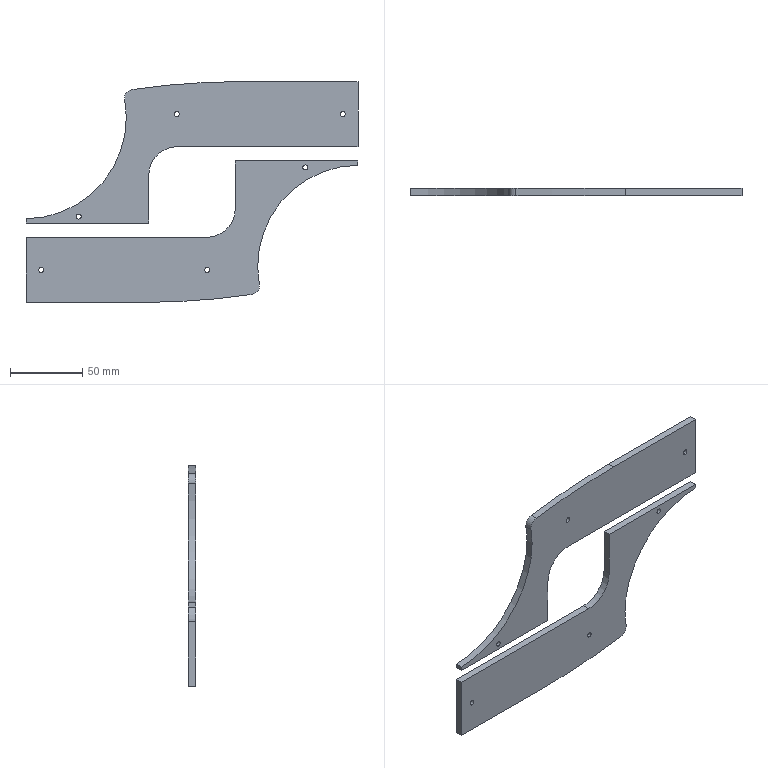CAM job | Mastercam | mm | 4 operations | part box 230 x 5 x 153
1. Contour (Ramp) | 3 - 3 平铣刀
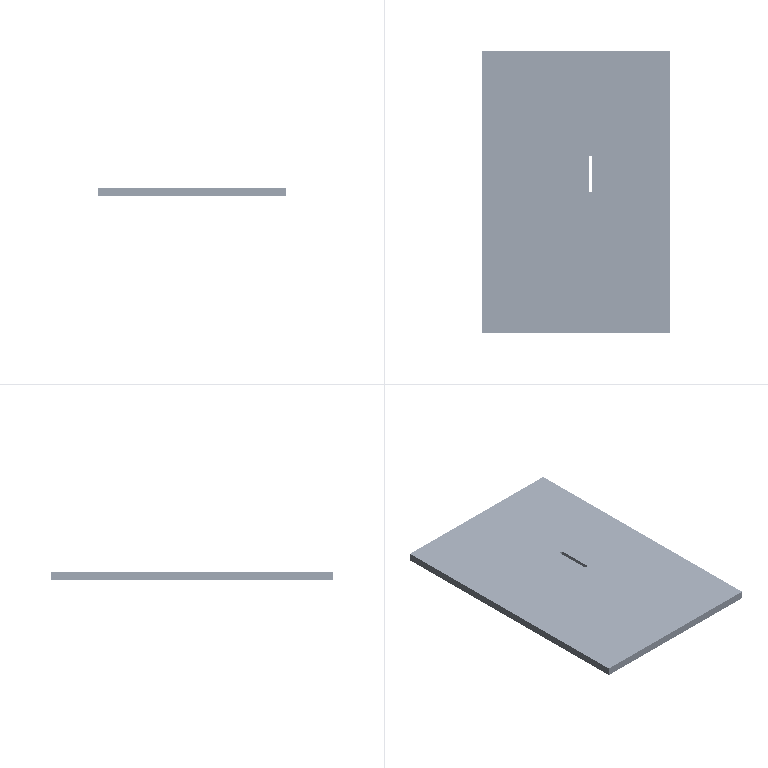2. Contour (2D) | 3 - 3 平铣刀
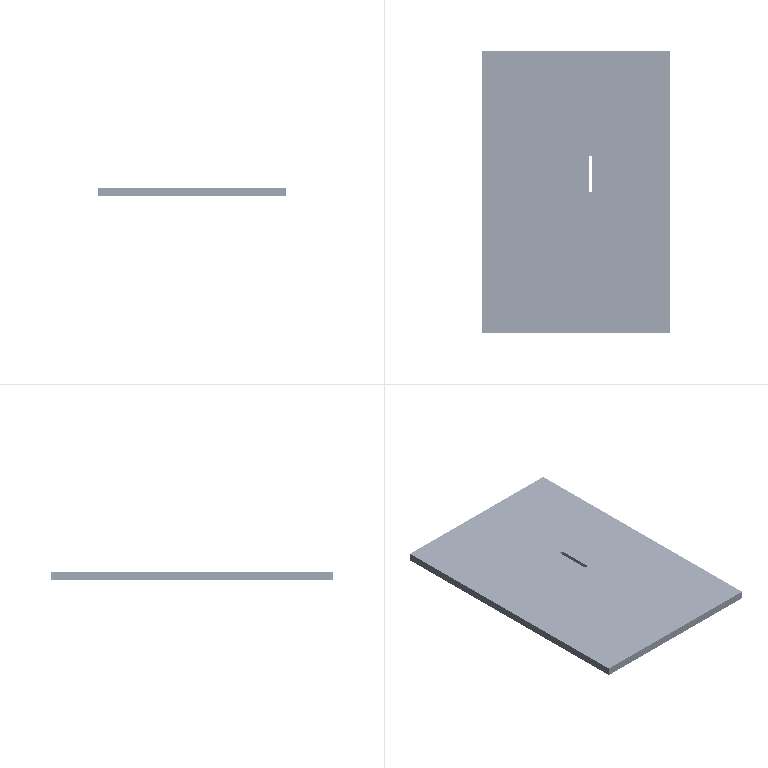3. Drill/Counterbore | 7 - 4 倒角刀
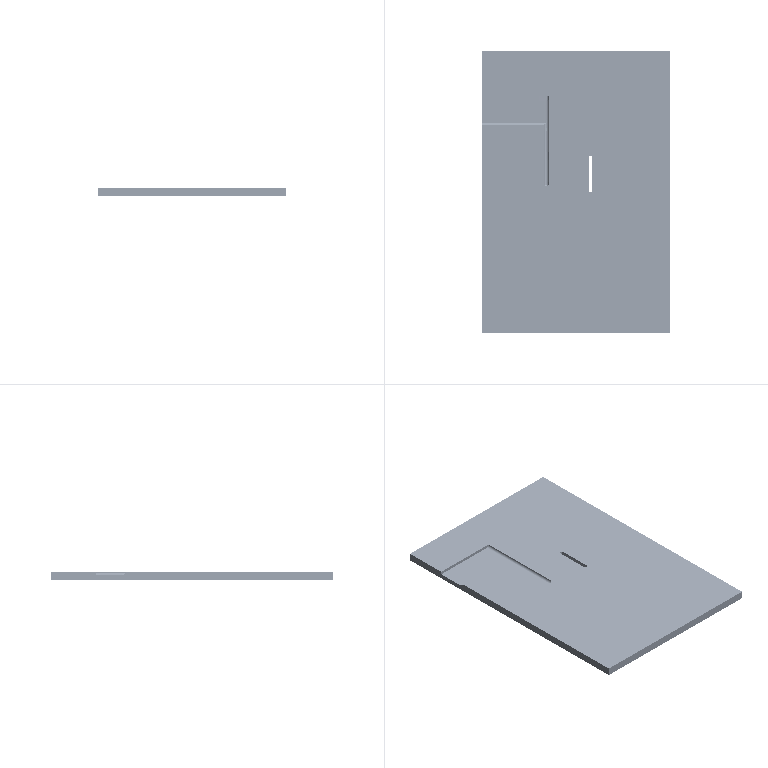4. Contour (2D chamfer) | 7 - 4 倒角刀